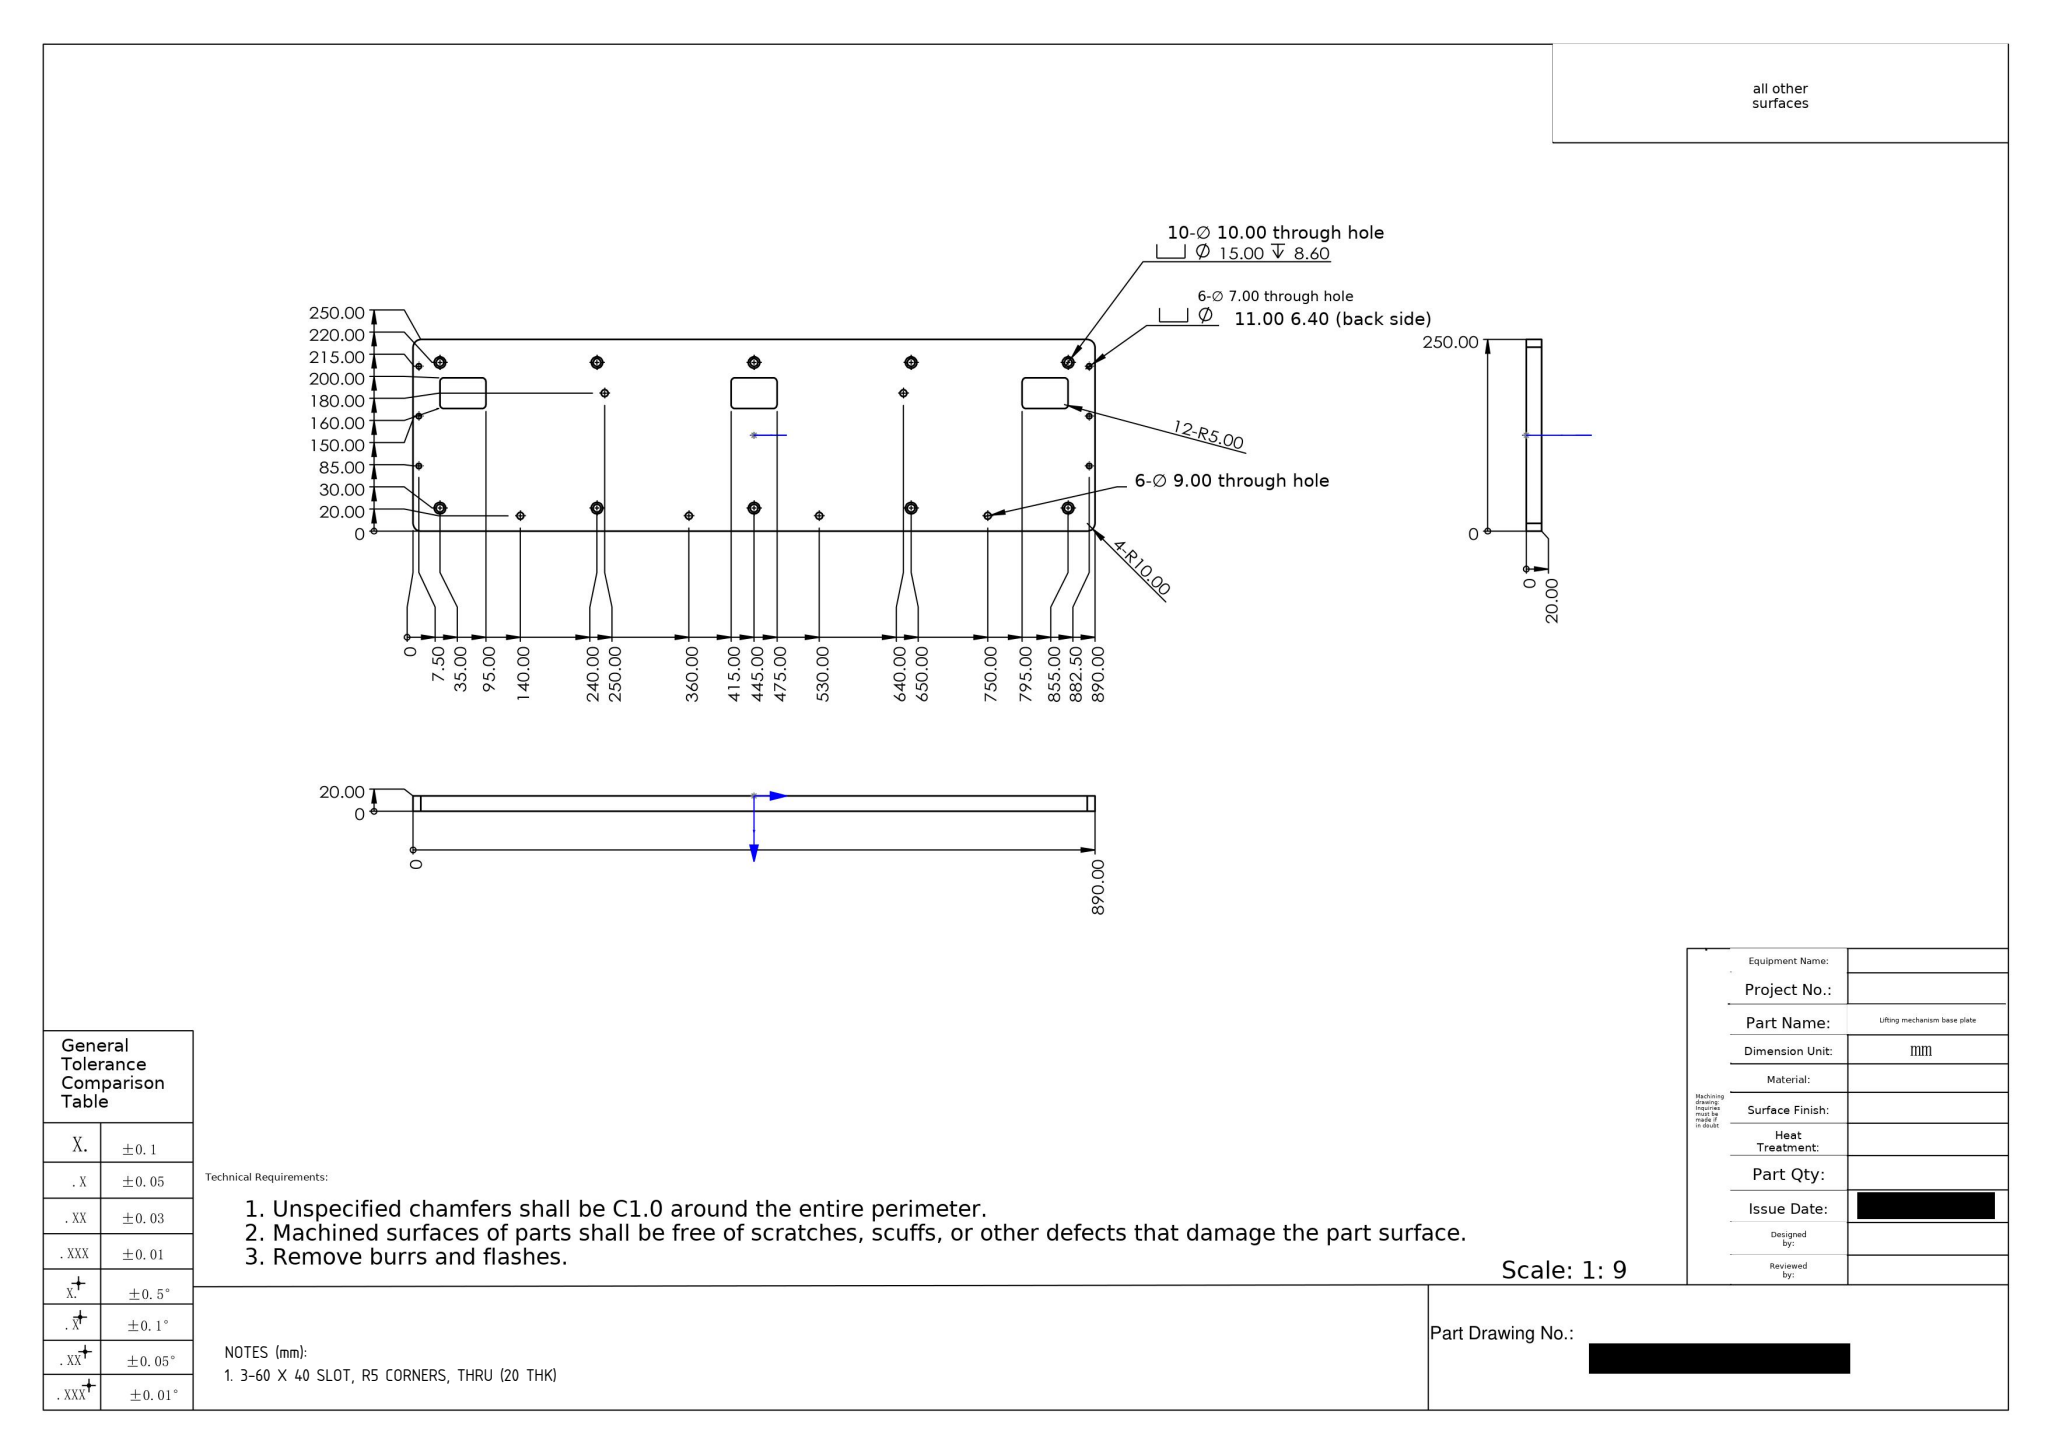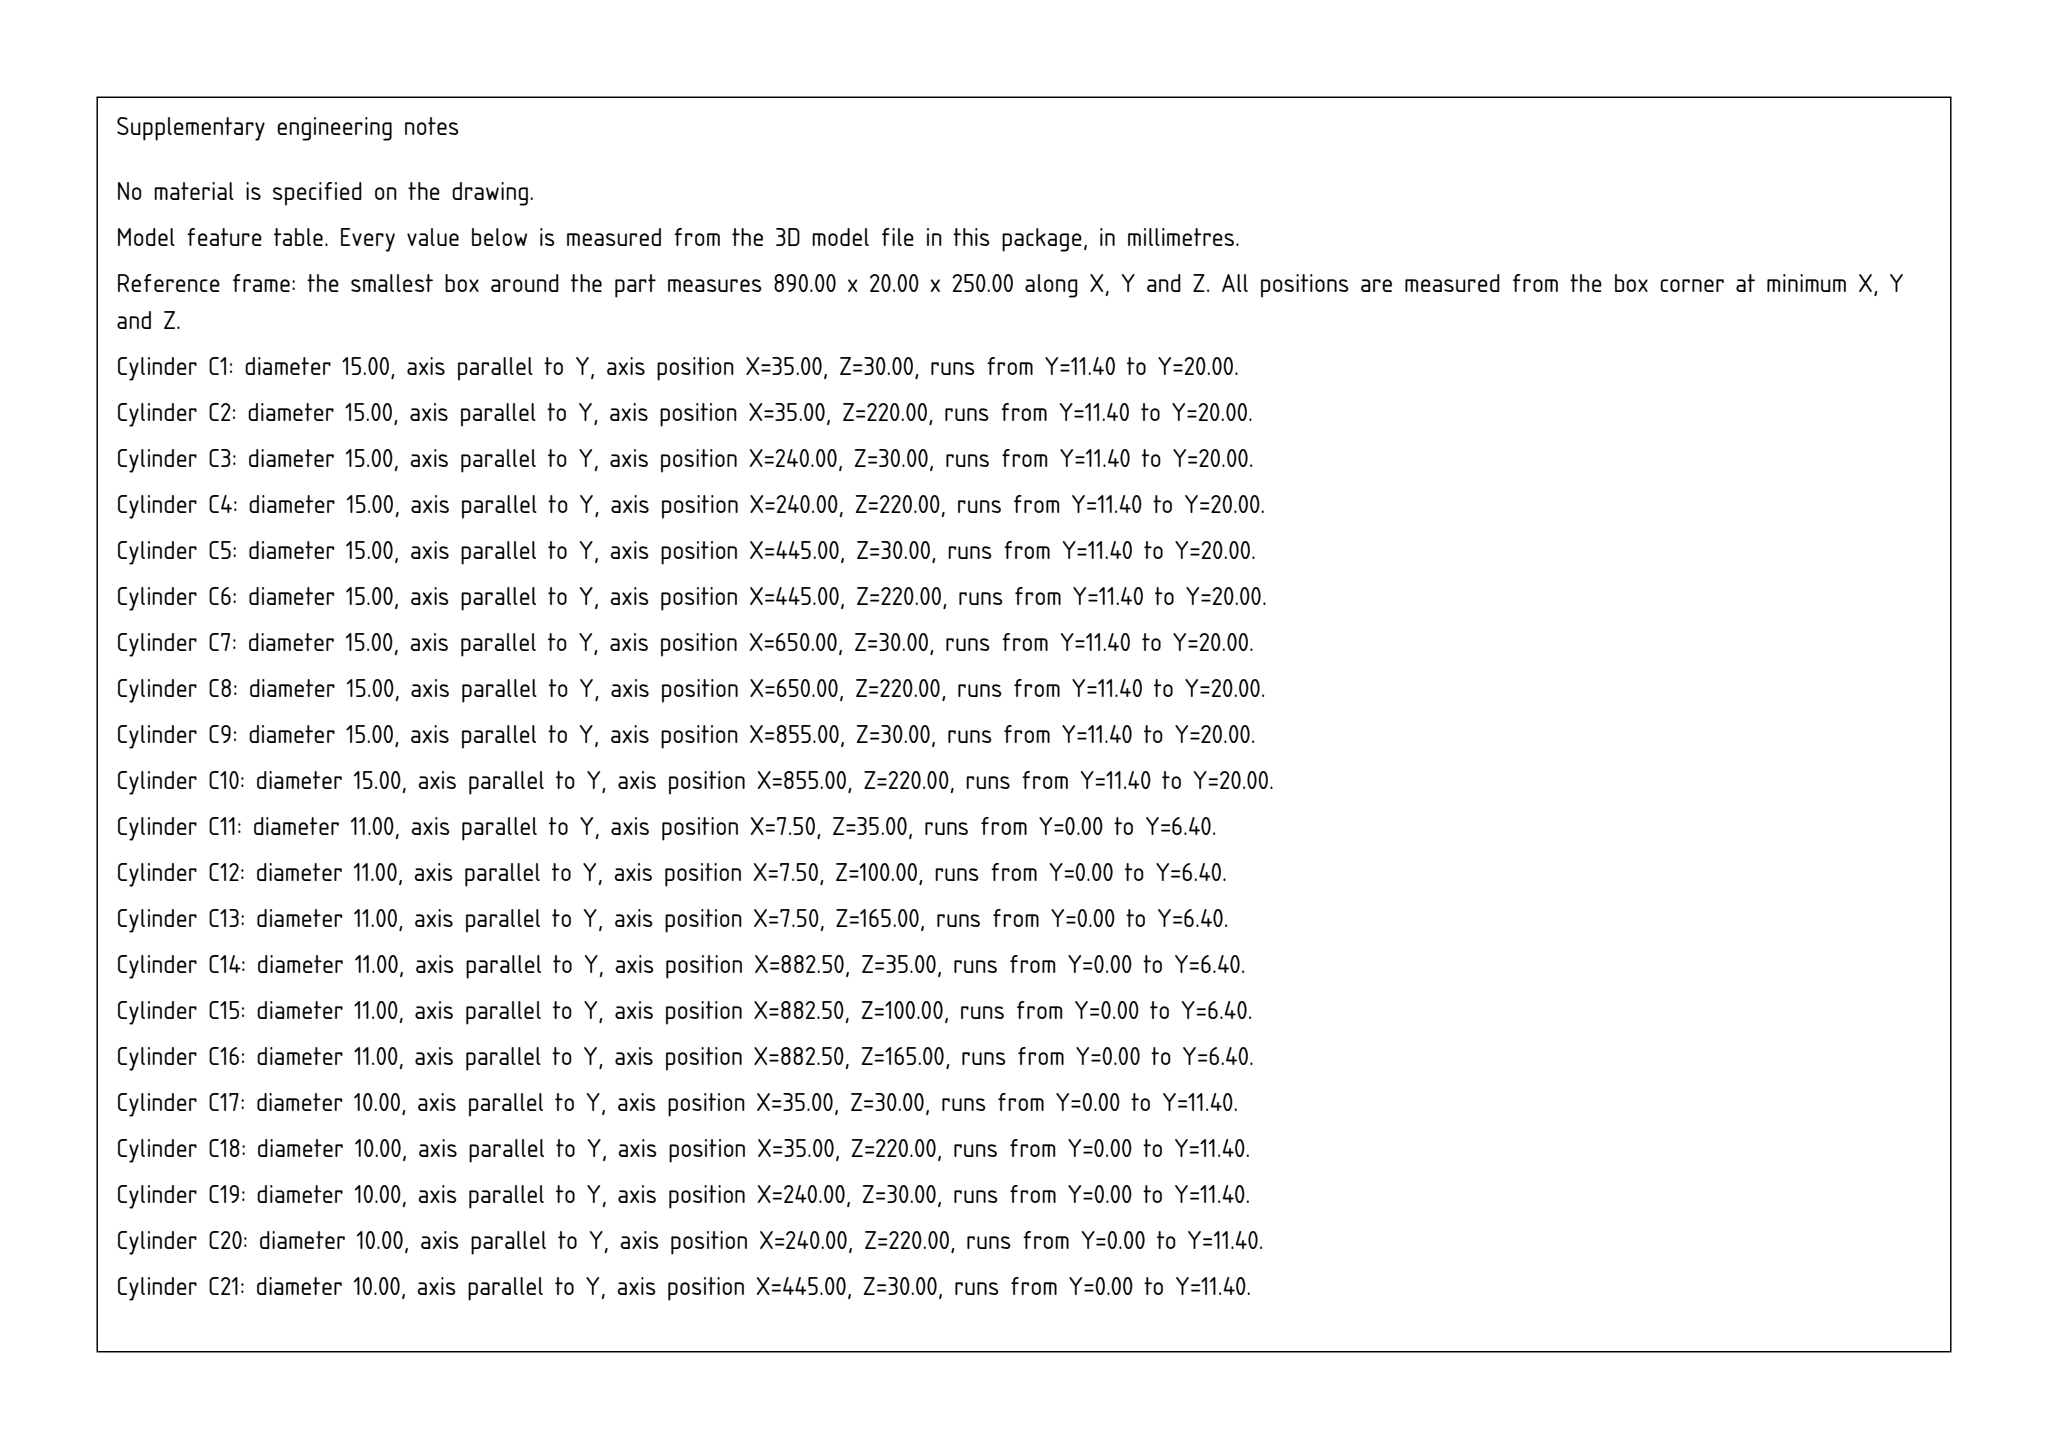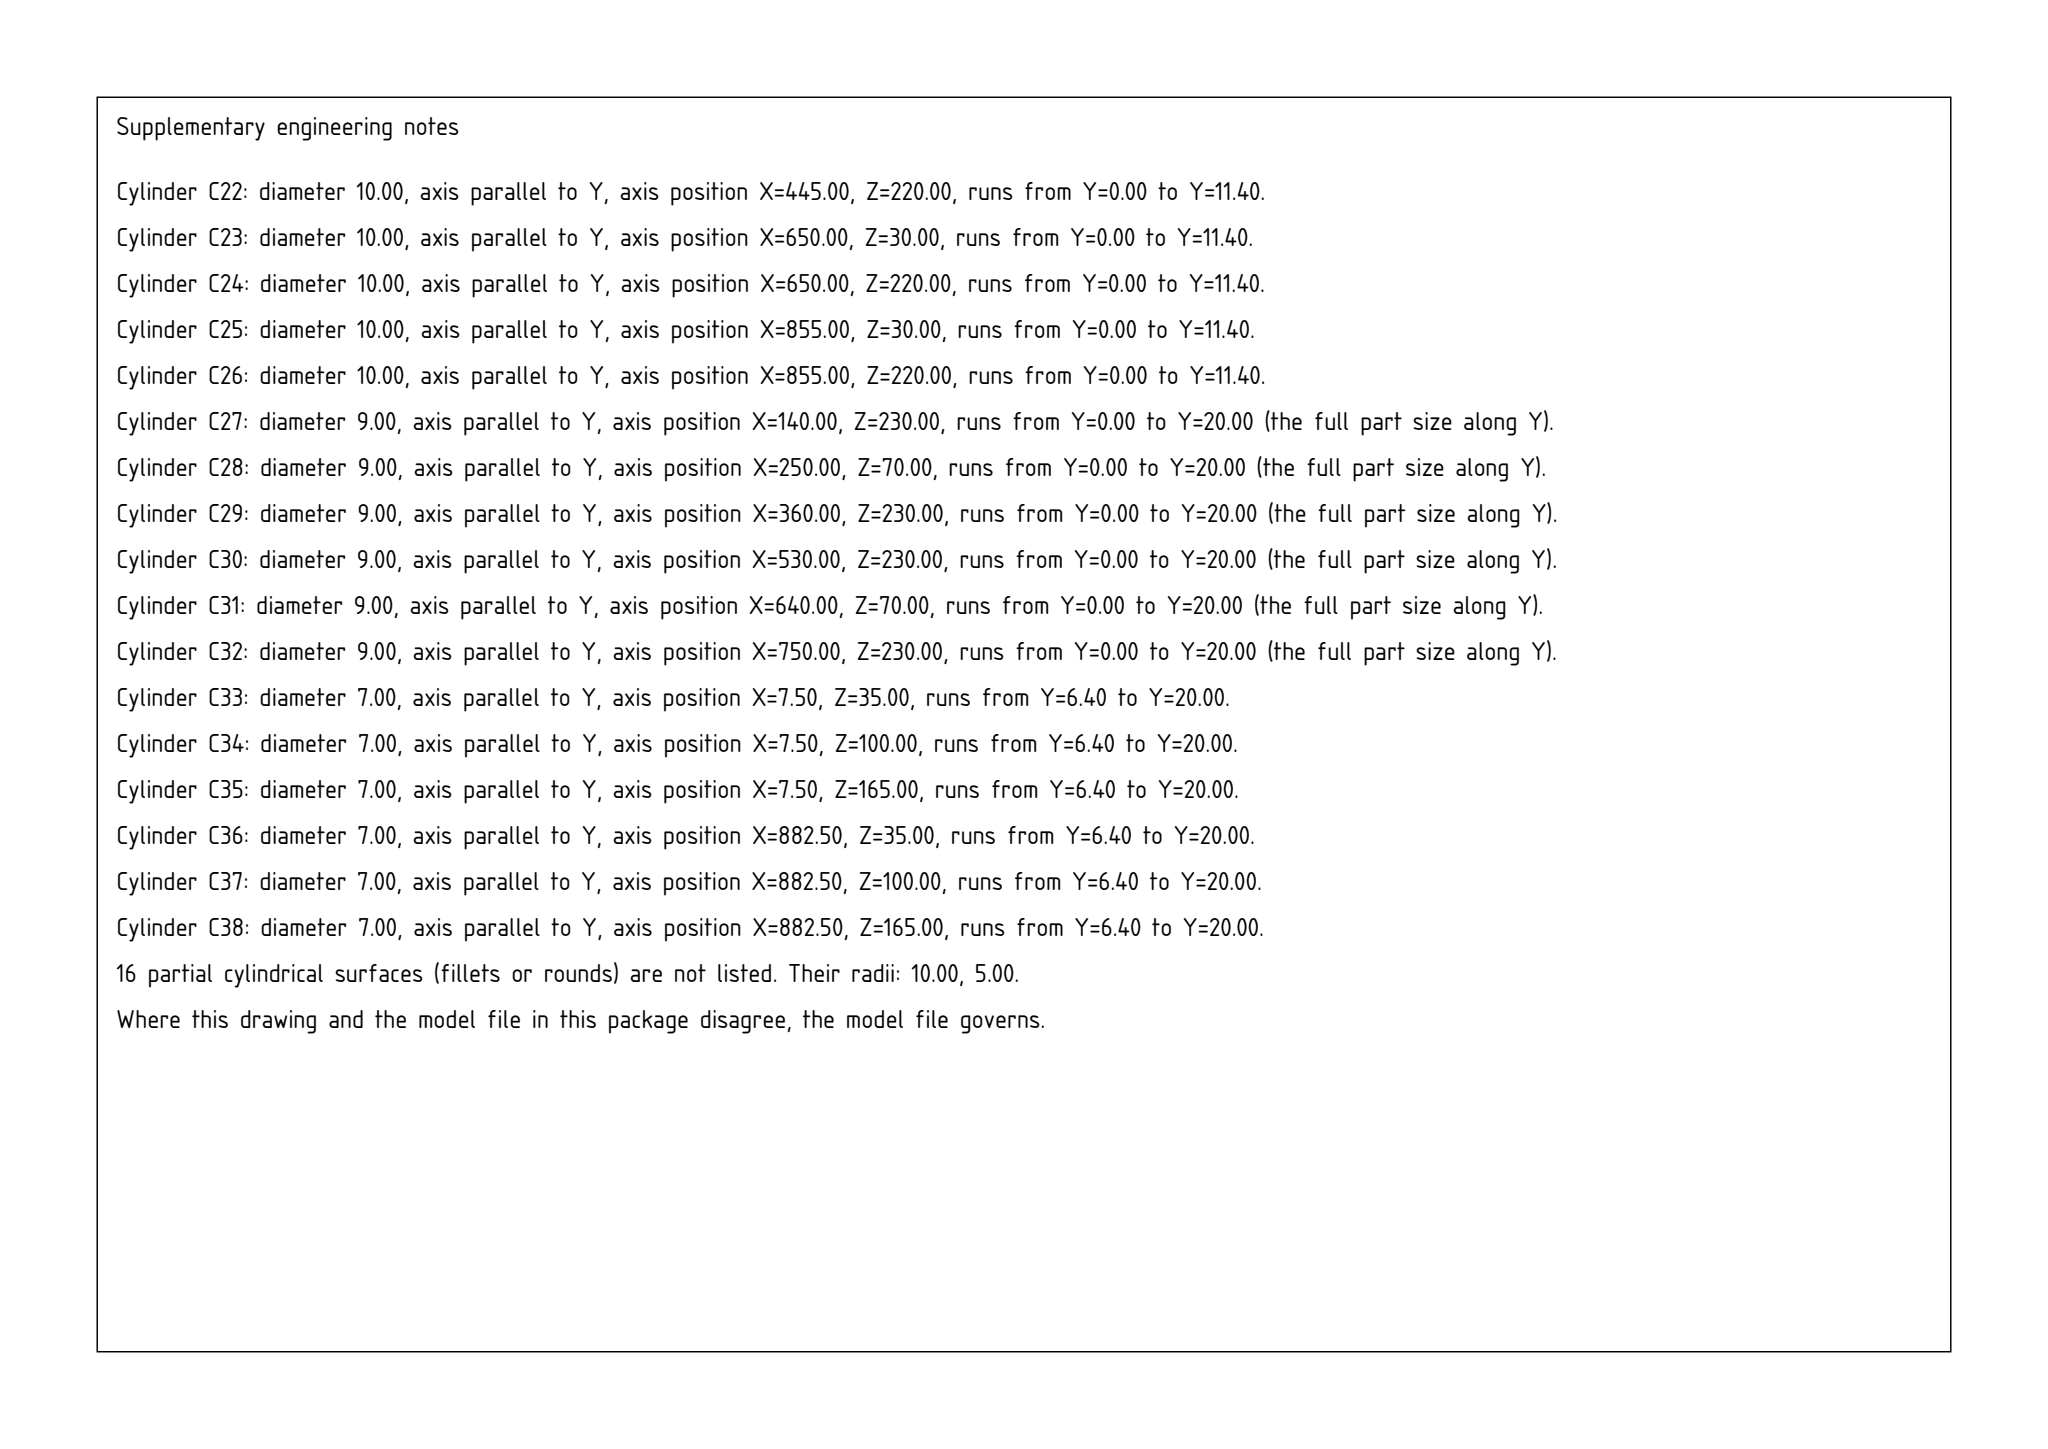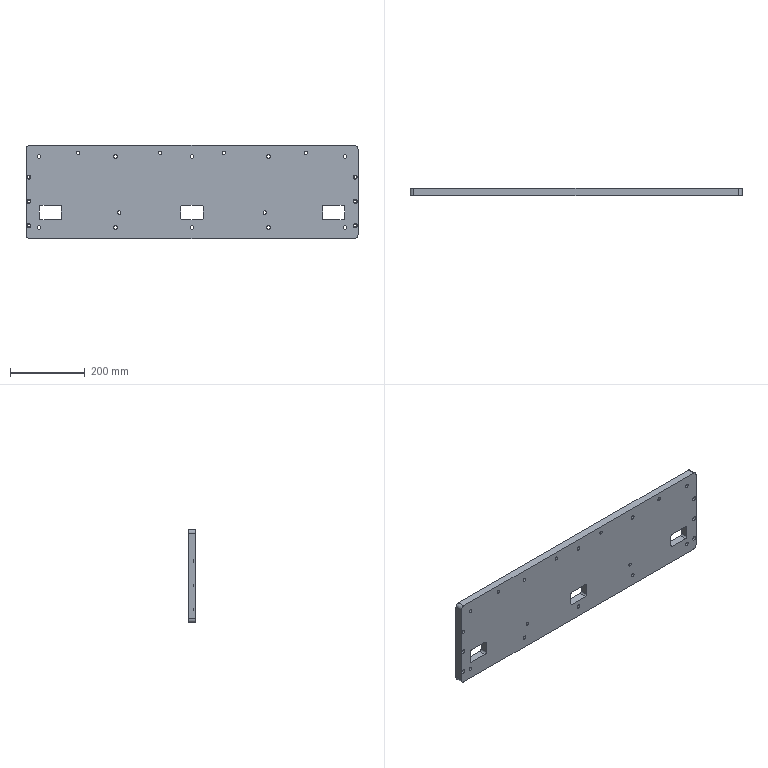Part | SolidWorks | mm | 1 solid | 126 faces | box 890 x 20 x 250 mm | volume 4266996 mm3 | cylinder 92 | plane 34 | commonest cylinder face diameters 10 x32 15 x20 11 x12 7 x12 9 x12 20 x4
Drawing notes:
3-60 X 40 SLOT, R5 CORNERS, THRU (20 THK) | from the solid: x planes 35/95, 415/475, 795/855 with z planes 50/90; plate y 0-20 thk, slot faces span full thickness
build123d program:
from build123d import *

# Parameters (mm, degrees)
SKETCH1_W                                       = 890
SKETCH1_H                                       = 250
BOSS_EXTRUDE1_DEPTH                             = 20
M8_CLEARANCE_HOLE2_D                            = 9
FILLET1_R                                       = 10
SKETCH14_W                                      = 60
SKETCH14_H                                      = 40
CUT_EXTRUDE1_DEPTH                              = 463.655
FILLET2_R                                       = 5
M8_HEX_SOCKET_HEAD_CAP_SCREW_CBORE1_D           = 10
M8_HEX_SOCKET_HEAD_CAP_SCREW_CBORE1_CBORE_D     = 15
M8_HEX_SOCKET_HEAD_CAP_SCREW_CBORE1_CBORE_DEPTH = 8.6
M6_HEX_SOCKET_HEAD_CAP_SCREW_CBORE1_D           = 7
M6_HEX_SOCKET_HEAD_CAP_SCREW_CBORE1_CBORE_D     = 11
M6_HEX_SOCKET_HEAD_CAP_SCREW_CBORE1_CBORE_DEPTH = 6.4


with BuildPart() as part:
    # Sketch1 → Boss-Extrude1 (new body)
    with BuildSketch(Plane(origin=(0, 0, 0), x_dir=(1, 0, 0), z_dir=(0, 1, 0))):
        Rectangle(SKETCH1_W, SKETCH1_H)
    extrude(amount=BOSS_EXTRUDE1_DEPTH)

    # M8 Clearance Hole2 (through all)
    with Locations(Plane(origin=(0, 20, 0), x_dir=(1, 0, 0), z_dir=(0, 1, 0))):
        with Locations((195, 55), (-195, 55), (-305, -105), (-85, -105), (85, -105), (305, -105)):
            Hole(M8_CLEARANCE_HOLE2_D / 2)

    # Fillet1
    fillet1_edges = [part.edges().sort_by_distance(p)[0] for p in [
        (-445, 10, -125),
        (445, 10, -125),
        (445, 10, 125),
        (-445, 10, 125),
    ]]
    fillet(fillet1_edges, radius=FILLET1_R)

    # Sketch14 → Cut-Extrude1 (cut, through all)
    with BuildSketch(Plane(origin=(0, 20, 0), x_dir=(1, 0, 0), z_dir=(0, 1, 0))):
        with Locations((-380, 55)):
            Rectangle(SKETCH14_W, SKETCH14_H)
        with Locations((0, 55)):
            Rectangle(SKETCH14_W, SKETCH14_H)
        with Locations((380, 55)):
            Rectangle(SKETCH14_W, SKETCH14_H)
    extrude(amount=-CUT_EXTRUDE1_DEPTH, mode=Mode.SUBTRACT)

    # Fillet2
    fillet2_edges = [part.edges().sort_by_distance(p)[0] for p in [
        (350, 10, -35),
        (350, 10, -75),
        (410, 10, -75),
        (410, 10, -35),
        (-410, 10, -35),
        (-410, 10, -75),
        (-350, 10, -75),
        (-350, 10, -35),
        (-30, 10, -35),
        (-30, 10, -75),
        (30, 10, -75),
        (30, 10, -35),
    ]]
    fillet(fillet2_edges, radius=FILLET2_R)

    # M8 Hex Socket Head Cap Screw CBORE1 (through all)
    with Locations(Plane(origin=(0, 20, 0), x_dir=(1, 0, 0), z_dir=(0, 1, 0))):
        with Locations((-410, -95), (-205, -95), (0, -95), (205, -95), (410, -95)):
            m8_hex_socket_head_cap_screw_cbore1 = CounterBoreHole(M8_HEX_SOCKET_HEAD_CAP_SCREW_CBORE1_D / 2, M8_HEX_SOCKET_HEAD_CAP_SCREW_CBORE1_CBORE_D / 2, M8_HEX_SOCKET_HEAD_CAP_SCREW_CBORE1_CBORE_DEPTH)

    # Mirror1: M8 Hex Socket Head Cap Screw CBORE1 across plane
    add(m8_hex_socket_head_cap_screw_cbore1.mirror(Plane.XY), mode=Mode.SUBTRACT)

    # M6 Hex Socket Head Cap Screw CBORE1 (through all)
    with Locations(Plane(origin=(0, 0, 0), x_dir=(-1, 0, 0), z_dir=(0, -1, 0))):
        with Locations((-437.5, 90), (-437.5, 25), (-437.5, -40), (437.5, -40), (437.5, 25), (437.5, 90)):
            CounterBoreHole(M6_HEX_SOCKET_HEAD_CAP_SCREW_CBORE1_D / 2, M6_HEX_SOCKET_HEAD_CAP_SCREW_CBORE1_CBORE_D / 2, M6_HEX_SOCKET_HEAD_CAP_SCREW_CBORE1_CBORE_DEPTH)


solid = part.part